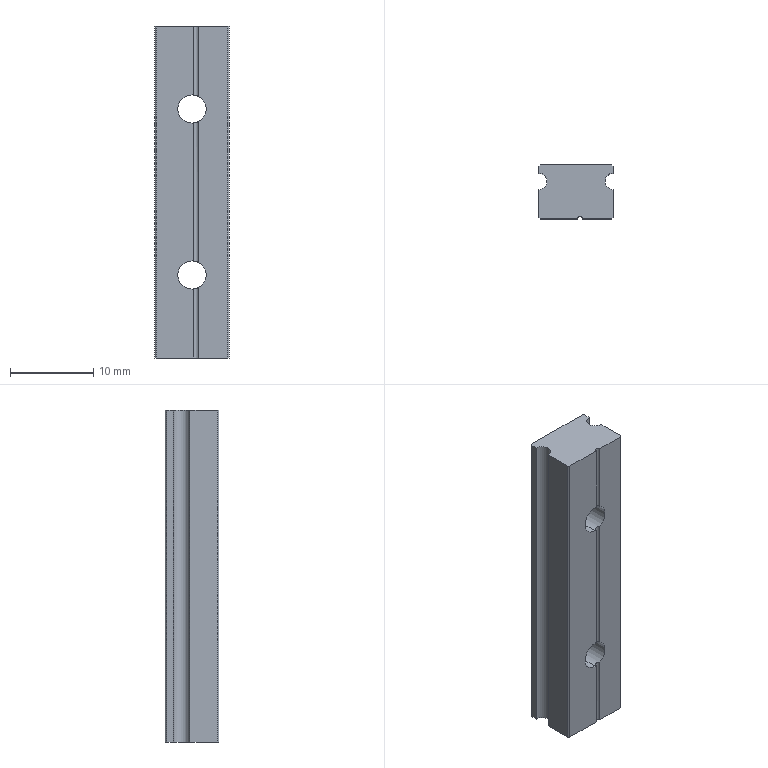Component | SolidWorks | MGN9C1R55Z0C(E=7.5)-10 | 1 solid | 29 faces | box 9 x 6.5 x 40 mm | volume 1924 mm3 | plane 15 | cylinder 14 | commonest cylinder face diameters 6.5 x4 3.4 x4 2 x3 0.6 x3
STEP:
#1=COLOUR_RGB('',0.7922,0.8196,0.9333);
#2=FILL_AREA_STYLE_COLOUR('',#1);
#3=FILL_AREA_STYLE('',(#2));
#4=SURFACE_STYLE_FILL_AREA(#3);
#5=SURFACE_SIDE_STYLE('',(#4));
#6=SURFACE_STYLE_USAGE(.BOTH.,#5);
#7=PRESENTATION_STYLE_ASSIGNMENT((#6));
#8=CARTESIAN_POINT('',(-1.043,-0.6806,-4.824));
#9=VERTEX_POINT('',#8);
#10=CARTESIAN_POINT('',(-1.043,-0.6806,-4.569));
#11=VERTEX_POINT('',#10);
#12=CARTESIAN_POINT('',(-1.043,-0.6806,-4.697));
#13=DIRECTION('',(0.,1.,0.));
#14=DIRECTION('',(0.,0.,1.));
#15=AXIS2_PLACEMENT_3D('',#12,#13,#14);
#16=CIRCLE('',#15,0.128);
#17=EDGE_CURVE('',#9,#11,#16,.T.);
#18=ORIENTED_EDGE('',*,*,#17,.F.);
#19=CARTESIAN_POINT('',(-1.043,-0.5468,-4.824));
#20=VERTEX_POINT('',#19);
#21=CARTESIAN_POINT('',(-1.043,-0.5468,-4.824));
#22=DIRECTION('',(0.,1.,0.));
#23=VECTOR('',#22,39.37);
#24=LINE('',#21,#23);
#25=EDGE_CURVE('',#9,#20,#24,.T.);
#26=ORIENTED_EDGE('',*,*,#25,.T.);
#27=CARTESIAN_POINT('',(-1.043,-0.5468,-4.569));
#28=VERTEX_POINT('',#27);
#29=CARTESIAN_POINT('',(-1.043,-0.5468,-4.697));
#30=DIRECTION('',(0.,1.,0.));
#31=DIRECTION('',(0.,0.,1.));
#32=AXIS2_PLACEMENT_3D('',#29,#30,#31);
#33=CIRCLE('',#32,0.128);
#34=EDGE_CURVE('',#20,#28,#33,.T.);
#35=ORIENTED_EDGE('',*,*,#34,.T.);
#36=CARTESIAN_POINT('',(-1.043,-0.5468,-4.569));
#37=DIRECTION('',(0.,1.,0.));
#38=VECTOR('',#37,39.37);
#39=LINE('',#36,#38);
#40=EDGE_CURVE('',#11,#28,#39,.T.);
#41=ORIENTED_EDGE('',*,*,#40,.F.);
#42=EDGE_LOOP('',(#18,#26,#35,#41));
#43=FACE_OUTER_BOUND('',#42,.T.);
#44=CARTESIAN_POINT('',(-1.043,-0.5468,-4.697));
#45=DIRECTION('',(0.,1.,0.));
#46=DIRECTION('',(0.,0.,1.));
#47=AXIS2_PLACEMENT_3D('',#44,#45,#46);
#48=CYLINDRICAL_SURFACE('',#47,0.128);
#49=ADVANCED_FACE('',(#43),#48,.F.);
#50=CARTESIAN_POINT('',(-1.043,-0.8027,-4.763));
#51=VERTEX_POINT('',#50);
#52=CARTESIAN_POINT('',(-1.043,-0.8027,-4.63));
#53=VERTEX_POINT('',#52);
#54=CARTESIAN_POINT('',(-1.043,-0.8027,-4.697));
#55=DIRECTION('',(-0.,1.,0.));
#56=DIRECTION('',(-1.,0.,0.));
#57=AXIS2_PLACEMENT_3D('',#54,#55,#56);
#58=CIRCLE('',#57,0.06693);
#59=EDGE_CURVE('',#51,#53,#58,.T.);
#60=ORIENTED_EDGE('',*,*,#59,.F.);
#61=CARTESIAN_POINT('',(-1.043,-0.6806,-4.763));
#62=VERTEX_POINT('',#61);
#63=CARTESIAN_POINT('',(-1.043,-0.5468,-4.763));
#64=DIRECTION('',(0.,1.,0.));
#65=VECTOR('',#64,39.37);
#66=LINE('',#63,#65);
#67=EDGE_CURVE('',#51,#62,#66,.T.);
#68=ORIENTED_EDGE('',*,*,#67,.T.);
#69=CARTESIAN_POINT('',(-1.043,-0.6806,-4.63));
#70=VERTEX_POINT('',#69);
#71=CARTESIAN_POINT('',(-1.043,-0.6806,-4.697));
#72=DIRECTION('',(0.,1.,0.));
#73=DIRECTION('',(0.,0.,1.));
#74=AXIS2_PLACEMENT_3D('',#71,#72,#73);
#75=CIRCLE('',#74,0.06693);
#76=EDGE_CURVE('',#62,#70,#75,.T.);
#77=ORIENTED_EDGE('',*,*,#76,.T.);
#78=CARTESIAN_POINT('',(-1.043,-0.5468,-4.63));
#79=DIRECTION('',(0.,1.,0.));
#80=VECTOR('',#79,39.37);
#81=LINE('',#78,#80);
#82=EDGE_CURVE('',#53,#70,#81,.T.);
#83=ORIENTED_EDGE('',*,*,#82,.F.);
#84=EDGE_LOOP('',(#60,#68,#77,#83));
#85=FACE_OUTER_BOUND('',#84,.T.);
#86=CARTESIAN_POINT('',(-1.043,-0.5468,-4.697));
#87=DIRECTION('',(0.,1.,0.));
#88=DIRECTION('',(0.,0.,1.));
#89=AXIS2_PLACEMENT_3D('',#86,#87,#88);
#90=CYLINDRICAL_SURFACE('',#89,0.06693);
#91=ADVANCED_FACE('',(#85),#90,.F.);
#92=CARTESIAN_POINT('',(-1.043,-0.6806,-4.037));
#93=VERTEX_POINT('',#92);
#94=CARTESIAN_POINT('',(-1.043,-0.6806,-3.781));
#95=VERTEX_POINT('',#94);
#96=CARTESIAN_POINT('',(-1.043,-0.6806,-3.909));
#97=DIRECTION('',(0.,1.,0.));
#98=DIRECTION('',(0.,0.,1.));
#99=AXIS2_PLACEMENT_3D('',#96,#97,#98);
#100=CIRCLE('',#99,0.128);
#101=EDGE_CURVE('',#93,#95,#100,.T.);
#102=ORIENTED_EDGE('',*,*,#101,.F.);
#103=CARTESIAN_POINT('',(-1.043,-0.5468,-4.037));
#104=VERTEX_POINT('',#103);
#105=CARTESIAN_POINT('',(-1.043,-0.5468,-4.037));
#106=DIRECTION('',(0.,1.,0.));
#107=VECTOR('',#106,39.37);
#108=LINE('',#105,#107);
#109=EDGE_CURVE('',#93,#104,#108,.T.);
#110=ORIENTED_EDGE('',*,*,#109,.T.);
#111=CARTESIAN_POINT('',(-1.043,-0.5468,-3.781));
#112=VERTEX_POINT('',#111);
#113=CARTESIAN_POINT('',(-1.043,-0.5468,-3.909));
#114=DIRECTION('',(0.,1.,0.));
#115=DIRECTION('',(0.,0.,1.));
#116=AXIS2_PLACEMENT_3D('',#113,#114,#115);
#117=CIRCLE('',#116,0.128);
#118=EDGE_CURVE('',#104,#112,#117,.T.);
#119=ORIENTED_EDGE('',*,*,#118,.T.);
#120=CARTESIAN_POINT('',(-1.043,-0.5468,-3.781));
#121=DIRECTION('',(0.,1.,0.));
#122=VECTOR('',#121,39.37);
#123=LINE('',#120,#122);
#124=EDGE_CURVE('',#95,#112,#123,.T.);
#125=ORIENTED_EDGE('',*,*,#124,.F.);
#126=EDGE_LOOP('',(#102,#110,#119,#125));
#127=FACE_OUTER_BOUND('',#126,.T.);
#128=CARTESIAN_POINT('',(-1.043,-0.5468,-3.909));
#129=DIRECTION('',(0.,1.,0.));
#130=DIRECTION('',(0.,0.,1.));
#131=AXIS2_PLACEMENT_3D('',#128,#129,#130);
#132=CYLINDRICAL_SURFACE('',#131,0.128);
#133=ADVANCED_FACE('',(#127),#132,.F.);
#134=CARTESIAN_POINT('',(-1.043,-0.8027,-3.976));
#135=VERTEX_POINT('',#134);
#136=CARTESIAN_POINT('',(-1.043,-0.8027,-3.842));
#137=VERTEX_POINT('',#136);
#138=CARTESIAN_POINT('',(-1.043,-0.8027,-3.909));
#139=DIRECTION('',(-0.,1.,0.));
#140=DIRECTION('',(-1.,0.,0.));
#141=AXIS2_PLACEMENT_3D('',#138,#139,#140);
#142=CIRCLE('',#141,0.06693);
#143=EDGE_CURVE('',#135,#137,#142,.T.);
#144=ORIENTED_EDGE('',*,*,#143,.F.);
#145=CARTESIAN_POINT('',(-1.043,-0.6806,-3.976));
#146=VERTEX_POINT('',#145);
#147=CARTESIAN_POINT('',(-1.043,-0.5468,-3.976));
#148=DIRECTION('',(0.,1.,0.));
#149=VECTOR('',#148,39.37);
#150=LINE('',#147,#149);
#151=EDGE_CURVE('',#135,#146,#150,.T.);
#152=ORIENTED_EDGE('',*,*,#151,.T.);
#153=CARTESIAN_POINT('',(-1.043,-0.6806,-3.842));
#154=VERTEX_POINT('',#153);
#155=CARTESIAN_POINT('',(-1.043,-0.6806,-3.909));
#156=DIRECTION('',(0.,1.,0.));
#157=DIRECTION('',(0.,0.,1.));
#158=AXIS2_PLACEMENT_3D('',#155,#156,#157);
#159=CIRCLE('',#158,0.06693);
#160=EDGE_CURVE('',#146,#154,#159,.T.);
#161=ORIENTED_EDGE('',*,*,#160,.T.);
#162=CARTESIAN_POINT('',(-1.043,-0.5468,-3.842));
#163=DIRECTION('',(0.,1.,0.));
#164=VECTOR('',#163,39.37);
#165=LINE('',#162,#164);
#166=EDGE_CURVE('',#137,#154,#165,.T.);
#167=ORIENTED_EDGE('',*,*,#166,.F.);
#168=EDGE_LOOP('',(#144,#152,#161,#167));
#169=FACE_OUTER_BOUND('',#168,.T.);
#170=CARTESIAN_POINT('',(-1.043,-0.5468,-3.909));
#171=DIRECTION('',(0.,1.,0.));
#172=DIRECTION('',(0.,0.,1.));
#173=AXIS2_PLACEMENT_3D('',#170,#171,#172);
#174=CYLINDRICAL_SURFACE('',#173,0.06693);
#175=ADVANCED_FACE('',(#169),#174,.F.);
#176=CARTESIAN_POINT('',(-0.8657,-0.5861,-3.515));
#177=VERTEX_POINT('',#176);
#178=CARTESIAN_POINT('',(-0.9051,-0.6255,-3.515));
#179=VERTEX_POINT('',#178);
#180=CARTESIAN_POINT('',(-0.8657,-0.6255,-3.515));
#181=DIRECTION('',(0.,0.,1.));
#182=DIRECTION('',(-1.,0.,0.));
#183=AXIS2_PLACEMENT_3D('',#180,#181,#182);
#184=CIRCLE('',#183,0.03937);
#185=EDGE_CURVE('',#177,#179,#184,.T.);
#186=ORIENTED_EDGE('',*,*,#185,.T.);
#187=CARTESIAN_POINT('',(-0.9051,-0.6255,-5.09));
#188=VERTEX_POINT('',#187);
#189=CARTESIAN_POINT('',(-0.9051,-0.6255,-3.515));
#190=DIRECTION('',(0.,0.,-1.));
#191=VECTOR('',#190,39.37);
#192=LINE('',#189,#191);
#193=EDGE_CURVE('',#179,#188,#192,.T.);
#194=ORIENTED_EDGE('',*,*,#193,.T.);
#195=CARTESIAN_POINT('',(-0.8657,-0.5861,-5.09));
#196=VERTEX_POINT('',#195);
#197=CARTESIAN_POINT('',(-0.8657,-0.6255,-5.09));
#198=DIRECTION('',(0.,0.,-1.));
#199=DIRECTION('',(1.,0.,0.));
#200=AXIS2_PLACEMENT_3D('',#197,#198,#199);
#201=CIRCLE('',#200,0.03937);
#202=EDGE_CURVE('',#188,#196,#201,.T.);
#203=ORIENTED_EDGE('',*,*,#202,.T.);
#204=CARTESIAN_POINT('',(-0.8657,-0.5861,-3.515));
#205=DIRECTION('',(0.,0.,-1.));
#206=VECTOR('',#205,39.37);
#207=LINE('',#204,#206);
#208=EDGE_CURVE('',#177,#196,#207,.T.);
#209=ORIENTED_EDGE('',*,*,#208,.F.);
#210=EDGE_LOOP('',(#186,#194,#203,#209));
#211=FACE_OUTER_BOUND('',#210,.T.);
#212=CARTESIAN_POINT('',(-0.8657,-0.6255,-3.515));
#213=DIRECTION('',(0.,0.,-1.));
#214=DIRECTION('',(-1.,0.,0.));
#215=AXIS2_PLACEMENT_3D('',#212,#213,#214);
#216=CYLINDRICAL_SURFACE('',#215,0.03937);
#217=ADVANCED_FACE('',(#211),#216,.F.);
#218=CARTESIAN_POINT('',(-1.035,-0.8027,-3.976));
#219=VERTEX_POINT('',#218);
#220=CARTESIAN_POINT('',(-1.035,-0.8027,-4.63));
#221=VERTEX_POINT('',#220);
#222=CARTESIAN_POINT('',(-1.035,-0.8027,-3.515));
#223=DIRECTION('',(0.,0.,-1.));
#224=VECTOR('',#223,39.37);
#225=LINE('',#222,#224);
#226=EDGE_CURVE('',#219,#221,#225,.T.);
#227=ORIENTED_EDGE('',*,*,#226,.T.);
#228=CARTESIAN_POINT('',(-1.011,-0.8027,-4.637));
#229=VERTEX_POINT('',#228);
#230=CARTESIAN_POINT('',(-1.035,-0.8027,-4.63));
#231=CARTESIAN_POINT('',(-1.035,-0.7995,-4.63));
#232=CARTESIAN_POINT('',(-1.034,-0.7963,-4.63));
#233=CARTESIAN_POINT('',(-1.029,-0.792,-4.631));
#234=CARTESIAN_POINT('',(-1.026,-0.7908,-4.632));
#235=CARTESIAN_POINT('',(-1.02,-0.7909,-4.634));
#236=CARTESIAN_POINT('',(-1.017,-0.7921,-4.635));
#237=CARTESIAN_POINT('',(-1.013,-0.7964,-4.637));
#238=CARTESIAN_POINT('',(-1.011,-0.7995,-4.637));
#239=CARTESIAN_POINT('',(-1.011,-0.8027,-4.637));
#240=B_SPLINE_CURVE_WITH_KNOTS('',3,(#230,#231,#232,#233,#234,#235,#236,#237,#238,#239),.UNSPECIFIED.,.F.,.F.,(4,2,2,2,4),(0.,0.0002407,0.0004815,0.0007222,0.0009629),.UNSPECIFIED.);
#241=EDGE_CURVE('',#221,#229,#240,.T.);
#242=ORIENTED_EDGE('',*,*,#241,.T.);
#243=CARTESIAN_POINT('',(-1.011,-0.8027,-3.968));
#244=VERTEX_POINT('',#243);
#245=CARTESIAN_POINT('',(-1.011,-0.8027,-3.515));
#246=DIRECTION('',(0.,0.,1.));
#247=VECTOR('',#246,39.37);
#248=LINE('',#245,#247);
#249=EDGE_CURVE('',#229,#244,#248,.T.);
#250=ORIENTED_EDGE('',*,*,#249,.T.);
#251=CARTESIAN_POINT('',(-1.011,-0.8027,-3.968));
#252=CARTESIAN_POINT('',(-1.011,-0.7995,-3.968));
#253=CARTESIAN_POINT('',(-1.013,-0.7964,-3.969));
#254=CARTESIAN_POINT('',(-1.017,-0.7922,-3.971));
#255=CARTESIAN_POINT('',(-1.02,-0.7909,-3.972));
#256=CARTESIAN_POINT('',(-1.026,-0.7908,-3.974));
#257=CARTESIAN_POINT('',(-1.029,-0.7919,-3.975));
#258=CARTESIAN_POINT('',(-1.034,-0.7963,-3.975));
#259=CARTESIAN_POINT('',(-1.035,-0.7995,-3.976));
#260=CARTESIAN_POINT('',(-1.035,-0.8027,-3.976));
#261=B_SPLINE_CURVE_WITH_KNOTS('',3,(#251,#252,#253,#254,#255,#256,#257,#258,#259,#260),.UNSPECIFIED.,.F.,.F.,(4,2,2,2,4),(0.,0.0002406,0.0004813,0.0007219,0.0009625),.UNSPECIFIED.);
#262=EDGE_CURVE('',#244,#219,#261,.T.);
#263=ORIENTED_EDGE('',*,*,#262,.T.);
#264=EDGE_LOOP('',(#227,#242,#250,#263));
#265=FACE_OUTER_BOUND('',#264,.T.);
#266=CARTESIAN_POINT('',(-1.023,-0.8027,-3.515));
#267=DIRECTION('',(0.,0.,-1.));
#268=DIRECTION('',(-1.,0.,0.));
#269=AXIS2_PLACEMENT_3D('',#266,#267,#268);
#270=CYLINDRICAL_SURFACE('',#269,0.01181);
#271=ADVANCED_FACE('',(#265),#270,.F.);
#272=CARTESIAN_POINT('',(-1.011,-0.8027,-5.09));
#273=VERTEX_POINT('',#272);
#274=CARTESIAN_POINT('',(-1.011,-0.8027,-4.756));
#275=VERTEX_POINT('',#274);
#276=CARTESIAN_POINT('',(-1.011,-0.8027,-3.515));
#277=DIRECTION('',(0.,0.,1.));
#278=VECTOR('',#277,39.37);
#279=LINE('',#276,#278);
#280=EDGE_CURVE('',#273,#275,#279,.T.);
#281=ORIENTED_EDGE('',*,*,#280,.T.);
#282=CARTESIAN_POINT('',(-1.035,-0.8027,-4.763));
#283=VERTEX_POINT('',#282);
#284=CARTESIAN_POINT('',(-1.011,-0.8027,-4.756));
#285=CARTESIAN_POINT('',(-1.011,-0.7995,-4.756));
#286=CARTESIAN_POINT('',(-1.013,-0.7964,-4.756));
#287=CARTESIAN_POINT('',(-1.017,-0.7922,-4.758));
#288=CARTESIAN_POINT('',(-1.02,-0.7909,-4.759));
#289=CARTESIAN_POINT('',(-1.026,-0.7908,-4.761));
#290=CARTESIAN_POINT('',(-1.029,-0.7919,-4.762));
#291=CARTESIAN_POINT('',(-1.034,-0.7963,-4.763));
#292=CARTESIAN_POINT('',(-1.035,-0.7995,-4.763));
#293=CARTESIAN_POINT('',(-1.035,-0.8027,-4.763));
#294=B_SPLINE_CURVE_WITH_KNOTS('',3,(#284,#285,#286,#287,#288,#289,#290,#291,#292,#293),.UNSPECIFIED.,.F.,.F.,(4,2,2,2,4),(0.,0.0002406,0.0004813,0.0007219,0.0009625),.UNSPECIFIED.);
#295=EDGE_CURVE('',#275,#283,#294,.T.);
#296=ORIENTED_EDGE('',*,*,#295,.T.);
#297=CARTESIAN_POINT('',(-1.035,-0.8027,-5.09));
#298=VERTEX_POINT('',#297);
#299=CARTESIAN_POINT('',(-1.035,-0.8027,-3.515));
#300=DIRECTION('',(0.,0.,-1.));
#301=VECTOR('',#300,39.37);
#302=LINE('',#299,#301);
#303=EDGE_CURVE('',#283,#298,#302,.T.);
#304=ORIENTED_EDGE('',*,*,#303,.T.);
#305=CARTESIAN_POINT('',(-1.023,-0.8027,-5.09));
#306=DIRECTION('',(0.,0.,-1.));
#307=DIRECTION('',(1.,0.,0.));
#308=AXIS2_PLACEMENT_3D('',#305,#306,#307);
#309=CIRCLE('',#308,0.01181);
#310=EDGE_CURVE('',#298,#273,#309,.T.);
#311=ORIENTED_EDGE('',*,*,#310,.T.);
#312=EDGE_LOOP('',(#281,#296,#304,#311));
#313=FACE_OUTER_BOUND('',#312,.T.);
#314=CARTESIAN_POINT('',(-1.023,-0.8027,-3.515));
#315=DIRECTION('',(0.,0.,-1.));
#316=DIRECTION('',(-1.,0.,0.));
#317=AXIS2_PLACEMENT_3D('',#314,#315,#316);
#318=CYLINDRICAL_SURFACE('',#317,0.01181);
#319=ADVANCED_FACE('',(#313),#318,.F.);
#320=CARTESIAN_POINT('',(-0.8736,-0.8027,-3.515));
#321=VERTEX_POINT('',#320);
#322=CARTESIAN_POINT('',(-0.8736,-0.8027,-5.09));
#323=VERTEX_POINT('',#322);
#324=CARTESIAN_POINT('',(-0.8736,-0.8027,-3.515));
#325=DIRECTION('',(0.,0.,-1.));
#326=VECTOR('',#325,39.37);
#327=LINE('',#324,#326);
#328=EDGE_CURVE('',#321,#323,#327,.T.);
#329=ORIENTED_EDGE('',*,*,#328,.T.);
#330=CARTESIAN_POINT('',(-0.8657,-0.7948,-5.09));
#331=VERTEX_POINT('',#330);
#332=CARTESIAN_POINT('',(-0.8736,-0.8027,-5.09));
#333=DIRECTION('',(0.7071,0.7071,0.));
#334=VECTOR('',#333,39.37);
#335=LINE('',#332,#334);
#336=EDGE_CURVE('',#323,#331,#335,.T.);
#337=ORIENTED_EDGE('',*,*,#336,.T.);
#338=CARTESIAN_POINT('',(-0.8657,-0.7948,-3.515));
#339=VERTEX_POINT('',#338);
#340=CARTESIAN_POINT('',(-0.8657,-0.7948,-3.515));
#341=DIRECTION('',(0.,0.,1.));
#342=VECTOR('',#341,39.37);
#343=LINE('',#340,#342);
#344=EDGE_CURVE('',#331,#339,#343,.T.);
#345=ORIENTED_EDGE('',*,*,#344,.T.);
#346=CARTESIAN_POINT('',(-0.8657,-0.7948,-3.515));
#347=DIRECTION('',(0.7071,0.7071,0.));
#348=VECTOR('',#347,39.37);
#349=LINE('',#346,#348);
#350=EDGE_CURVE('',#321,#339,#349,.T.);
#351=ORIENTED_EDGE('',*,*,#350,.F.);
#352=EDGE_LOOP('',(#329,#337,#345,#351));
#353=FACE_OUTER_BOUND('',#352,.T.);
#354=CARTESIAN_POINT('',(-0.8657,-0.7948,-3.515));
#355=DIRECTION('',(-0.7071,0.7071,0.));
#356=DIRECTION('',(-0.7071,-0.7071,0.));
#357=AXIS2_PLACEMENT_3D('',#354,#355,#356);
#358=PLANE('',#357);
#359=ADVANCED_FACE('',(#353),#358,.F.);
#360=CARTESIAN_POINT('',(-1.035,-0.8027,-3.515));
#361=VERTEX_POINT('',#360);
#362=CARTESIAN_POINT('',(-1.035,-0.8027,-3.843));
#363=VERTEX_POINT('',#362);
#364=CARTESIAN_POINT('',(-1.035,-0.8027,-3.515));
#365=DIRECTION('',(0.,0.,-1.));
#366=VECTOR('',#365,39.37);
#367=LINE('',#364,#366);
#368=EDGE_CURVE('',#361,#363,#367,.T.);
#369=ORIENTED_EDGE('',*,*,#368,.T.);
#370=CARTESIAN_POINT('',(-1.011,-0.8027,-3.85));
#371=VERTEX_POINT('',#370);
#372=CARTESIAN_POINT('',(-1.035,-0.8027,-3.843));
#373=CARTESIAN_POINT('',(-1.035,-0.7995,-3.843));
#374=CARTESIAN_POINT('',(-1.034,-0.7963,-3.843));
#375=CARTESIAN_POINT('',(-1.029,-0.792,-3.844));
#376=CARTESIAN_POINT('',(-1.026,-0.7908,-3.844));
#377=CARTESIAN_POINT('',(-1.02,-0.7909,-3.846));
#378=CARTESIAN_POINT('',(-1.017,-0.7921,-3.847));
#379=CARTESIAN_POINT('',(-1.013,-0.7964,-3.849));
#380=CARTESIAN_POINT('',(-1.011,-0.7995,-3.85));
#381=CARTESIAN_POINT('',(-1.011,-0.8027,-3.85));
#382=B_SPLINE_CURVE_WITH_KNOTS('',3,(#372,#373,#374,#375,#376,#377,#378,#379,#380,#381),.UNSPECIFIED.,.F.,.F.,(4,2,2,2,4),(0.,0.0002407,0.0004815,0.0007222,0.0009629),.UNSPECIFIED.);
#383=EDGE_CURVE('',#363,#371,#382,.T.);
#384=ORIENTED_EDGE('',*,*,#383,.T.);
#385=CARTESIAN_POINT('',(-1.011,-0.8027,-3.515));
#386=VERTEX_POINT('',#385);
#387=CARTESIAN_POINT('',(-1.011,-0.8027,-3.515));
#388=DIRECTION('',(0.,0.,1.));
#389=VECTOR('',#388,39.37);
#390=LINE('',#387,#389);
#391=EDGE_CURVE('',#371,#386,#390,.T.);
#392=ORIENTED_EDGE('',*,*,#391,.T.);
#393=CARTESIAN_POINT('',(-1.023,-0.8027,-3.515));
#394=DIRECTION('',(0.,0.,-1.));
#395=DIRECTION('',(-1.,0.,0.));
#396=AXIS2_PLACEMENT_3D('',#393,#394,#395);
#397=CIRCLE('',#396,0.01181);
#398=EDGE_CURVE('',#361,#386,#397,.T.);
#399=ORIENTED_EDGE('',*,*,#398,.F.);
#400=EDGE_LOOP('',(#369,#384,#392,#399));
#401=FACE_OUTER_BOUND('',#400,.T.);
#402=CARTESIAN_POINT('',(-1.023,-0.8027,-3.515));
#403=DIRECTION('',(0.,0.,-1.));
#404=DIRECTION('',(-1.,0.,0.));
#405=AXIS2_PLACEMENT_3D('',#402,#403,#404);
#406=CYLINDRICAL_SURFACE('',#405,0.01181);
#407=ADVANCED_FACE('',(#401),#406,.F.);
#408=CARTESIAN_POINT('',(-1.22,-0.7948,-3.515));
#409=VERTEX_POINT('',#408);
#410=CARTESIAN_POINT('',(-1.22,-0.7948,-5.09));
#411=VERTEX_POINT('',#410);
#412=CARTESIAN_POINT('',(-1.22,-0.7948,-3.515));
#413=DIRECTION('',(0.,0.,-1.));
#414=VECTOR('',#413,39.37);
#415=LINE('',#412,#414);
#416=EDGE_CURVE('',#409,#411,#415,.T.);
#417=ORIENTED_EDGE('',*,*,#416,.T.);
#418=CARTESIAN_POINT('',(-1.212,-0.8027,-5.09));
#419=VERTEX_POINT('',#418);
#420=CARTESIAN_POINT('',(-1.22,-0.7948,-5.09));
#421=DIRECTION('',(0.7071,-0.7071,0.));
#422=VECTOR('',#421,39.37);
#423=LINE('',#420,#422);
#424=EDGE_CURVE('',#411,#419,#423,.T.);
#425=ORIENTED_EDGE('',*,*,#424,.T.);
#426=CARTESIAN_POINT('',(-1.212,-0.8027,-3.515));
#427=VERTEX_POINT('',#426);
#428=CARTESIAN_POINT('',(-1.212,-0.8027,-3.515));
#429=DIRECTION('',(0.,0.,1.));
#430=VECTOR('',#429,39.37);
#431=LINE('',#428,#430);
#432=EDGE_CURVE('',#419,#427,#431,.T.);
#433=ORIENTED_EDGE('',*,*,#432,.T.);
#434=CARTESIAN_POINT('',(-1.212,-0.8027,-3.515));
#435=DIRECTION('',(0.7071,-0.7071,0.));
#436=VECTOR('',#435,39.37);
#437=LINE('',#434,#436);
#438=EDGE_CURVE('',#409,#427,#437,.T.);
#439=ORIENTED_EDGE('',*,*,#438,.F.);
#440=EDGE_LOOP('',(#417,#425,#433,#439));
#441=FACE_OUTER_BOUND('',#440,.T.);
#442=CARTESIAN_POINT('',(-1.212,-0.8027,-3.515));
#443=DIRECTION('',(0.7071,0.7071,0.));
#444=DIRECTION('',(-0.7071,0.7071,0.));
#445=AXIS2_PLACEMENT_3D('',#442,#443,#444);
#446=PLANE('',#445);
#447=ADVANCED_FACE('',(#441),#446,.F.);
#448=ORIENTED_EDGE('',*,*,#208,.T.);
#449=CARTESIAN_POINT('',(-0.8657,-0.5546,-5.09));
#450=VERTEX_POINT('',#449);
#451=CARTESIAN_POINT('',(-0.8657,-0.5861,-5.09));
#452=DIRECTION('',(0.,1.,0.));
#453=VECTOR('',#452,39.37);
#454=LINE('',#451,#453);
#455=EDGE_CURVE('',#196,#450,#454,.T.);
#456=ORIENTED_EDGE('',*,*,#455,.T.);
#457=CARTESIAN_POINT('',(-0.8657,-0.5546,-3.515));
#458=VERTEX_POINT('',#457);
#459=CARTESIAN_POINT('',(-0.8657,-0.5546,-3.515));
#460=DIRECTION('',(0.,0.,1.));
#461=VECTOR('',#460,39.37);
#462=LINE('',#459,#461);
#463=EDGE_CURVE('',#450,#458,#462,.T.);
#464=ORIENTED_EDGE('',*,*,#463,.T.);
#465=CARTESIAN_POINT('',(-0.8657,-0.5861,-3.515));
#466=DIRECTION('',(0.,1.,0.));
#467=VECTOR('',#466,39.37);
#468=LINE('',#465,#467);
#469=EDGE_CURVE('',#177,#458,#468,.T.);
#470=ORIENTED_EDGE('',*,*,#469,.F.);
#471=EDGE_LOOP('',(#448,#456,#464,#470));
#472=FACE_OUTER_BOUND('',#471,.T.);
#473=CARTESIAN_POINT('',(-0.8657,-0.5861,-3.515));
#474=DIRECTION('',(-1.,0.,0.));
#475=DIRECTION('',(0.,0.,1.));
#476=AXIS2_PLACEMENT_3D('',#473,#474,#475);
#477=PLANE('',#476);
#478=ADVANCED_FACE('',(#472),#477,.F.);
#479=CARTESIAN_POINT('',(-1.22,-0.5546,-3.515));
#480=VERTEX_POINT('',#479);
#481=CARTESIAN_POINT('',(-1.22,-0.5546,-5.09));
#482=VERTEX_POINT('',#481);
#483=CARTESIAN_POINT('',(-1.22,-0.5546,-3.515));
#484=DIRECTION('',(0.,0.,-1.));
#485=VECTOR('',#484,39.37);
#486=LINE('',#483,#485);
#487=EDGE_CURVE('',#480,#482,#486,.T.);
#488=ORIENTED_EDGE('',*,*,#487,.T.);
#489=CARTESIAN_POINT('',(-1.22,-0.5861,-5.09));
#490=VERTEX_POINT('',#489);
#491=CARTESIAN_POINT('',(-1.22,-0.5546,-5.09));
#492=DIRECTION('',(0.,-1.,0.));
#493=VECTOR('',#492,39.37);
#494=LINE('',#491,#493);
#495=EDGE_CURVE('',#482,#490,#494,.T.);
#496=ORIENTED_EDGE('',*,*,#495,.T.);
#497=CARTESIAN_POINT('',(-1.22,-0.5861,-3.515));
#498=VERTEX_POINT('',#497);
#499=CARTESIAN_POINT('',(-1.22,-0.5861,-3.515));
#500=DIRECTION('',(0.,0.,1.));
#501=VECTOR('',#500,39.37);
#502=LINE('',#499,#501);
#503=EDGE_CURVE('',#490,#498,#502,.T.);
#504=ORIENTED_EDGE('',*,*,#503,.T.);
#505=CARTESIAN_POINT('',(-1.22,-0.8027,-3.515));
#506=DIRECTION('',(0.,1.,0.));
#507=VECTOR('',#506,39.37);
#508=LINE('',#505,#507);
#509=EDGE_CURVE('',#498,#480,#508,.T.);
#510=ORIENTED_EDGE('',*,*,#509,.T.);
#511=EDGE_LOOP('',(#488,#496,#504,#510));
#512=FACE_OUTER_BOUND('',#511,.T.);
#513=CARTESIAN_POINT('',(-1.22,-0.5468,-3.515));
#514=DIRECTION('',(1.,0.,0.));
#515=DIRECTION('',(0.,0.,-1.));
#516=AXIS2_PLACEMENT_3D('',#513,#514,#515);
#517=PLANE('',#516);
#518=ADVANCED_FACE('',(#512),#517,.F.);
#519=ORIENTED_EDGE('',*,*,#344,.F.);
#520=CARTESIAN_POINT('',(-0.8657,-0.6649,-5.09));
#521=VERTEX_POINT('',#520);
#522=CARTESIAN_POINT('',(-0.8657,-0.7948,-5.09));
#523=DIRECTION('',(0.,1.,0.));
#524=VECTOR('',#523,39.37);
#525=LINE('',#522,#524);
#526=EDGE_CURVE('',#331,#521,#525,.T.);
#527=ORIENTED_EDGE('',*,*,#526,.T.);
#528=CARTESIAN_POINT('',(-0.8657,-0.6649,-3.515));
#529=VERTEX_POINT('',#528);
#530=CARTESIAN_POINT('',(-0.8657,-0.6649,-3.515));
#531=DIRECTION('',(0.,0.,1.));
#532=VECTOR('',#531,39.37);
#533=LINE('',#530,#532);
#534=EDGE_CURVE('',#521,#529,#533,.T.);
#535=ORIENTED_EDGE('',*,*,#534,.T.);
#536=CARTESIAN_POINT('',(-0.8657,-0.8027,-3.515));
#537=DIRECTION('',(0.,-1.,0.));
#538=VECTOR('',#537,39.37);
#539=LINE('',#536,#538);
#540=EDGE_CURVE('',#529,#339,#539,.T.);
#541=ORIENTED_EDGE('',*,*,#540,.T.);
#542=EDGE_LOOP('',(#519,#527,#535,#541));
#543=FACE_OUTER_BOUND('',#542,.T.);
#544=CARTESIAN_POINT('',(-0.8657,-0.8027,-3.515));
#545=DIRECTION('',(-1.,-0.,0.));
#546=DIRECTION('',(0.,-1.,0.));
#547=AXIS2_PLACEMENT_3D('',#544,#545,#546);
#548=PLANE('',#547);
#549=ADVANCED_FACE('',(#543),#548,.F.);
#550=ORIENTED_EDGE('',*,*,#249,.F.);
#551=CARTESIAN_POINT('',(-1.043,-0.8027,-4.697));
#552=DIRECTION('',(-0.,1.,0.));
#553=DIRECTION('',(-1.,0.,0.));
#554=AXIS2_PLACEMENT_3D('',#551,#552,#553);
#555=CIRCLE('',#554,0.06693);
#556=EDGE_CURVE('',#229,#275,#555,.T.);
#557=ORIENTED_EDGE('',*,*,#556,.T.);
#558=ORIENTED_EDGE('',*,*,#280,.F.);
#559=CARTESIAN_POINT('',(-1.011,-0.8027,-5.09));
#560=DIRECTION('',(1.,0.,0.));
#561=VECTOR('',#560,39.37);
#562=LINE('',#559,#561);
#563=EDGE_CURVE('',#273,#323,#562,.T.);
#564=ORIENTED_EDGE('',*,*,#563,.T.);
#565=ORIENTED_EDGE('',*,*,#328,.F.);
#566=CARTESIAN_POINT('',(-1.023,-0.8027,-3.515));
#567=DIRECTION('',(-1.,0.,0.));
#568=VECTOR('',#567,39.37);
#569=LINE('',#566,#568);
#570=EDGE_CURVE('',#321,#386,#569,.T.);
#571=ORIENTED_EDGE('',*,*,#570,.T.);
#572=ORIENTED_EDGE('',*,*,#391,.F.);
#573=CARTESIAN_POINT('',(-1.043,-0.8027,-3.909));
#574=DIRECTION('',(-0.,1.,0.));
#575=DIRECTION('',(-1.,0.,0.));
#576=AXIS2_PLACEMENT_3D('',#573,#574,#575);
#577=CIRCLE('',#576,0.06693);
#578=EDGE_CURVE('',#371,#244,#577,.T.);
#579=ORIENTED_EDGE('',*,*,#578,.T.);
#580=EDGE_LOOP('',(#550,#557,#558,#564,#565,#571,#572,#579));
#581=FACE_OUTER_BOUND('',#580,.T.);
#582=CARTESIAN_POINT('',(-1.011,-0.8027,-3.515));
#583=DIRECTION('',(-0.,1.,0.));
#584=DIRECTION('',(-1.,-0.,0.));
#585=AXIS2_PLACEMENT_3D('',#582,#583,#584);
#586=PLANE('',#585);
#587=ADVANCED_FACE('',(#581),#586,.F.);
#588=ORIENTED_EDGE('',*,*,#303,.F.);
#589=CARTESIAN_POINT('',(-1.043,-0.8027,-4.697));
#590=DIRECTION('',(-0.,1.,0.));
#591=DIRECTION('',(-1.,0.,0.));
#592=AXIS2_PLACEMENT_3D('',#589,#590,#591);
#593=CIRCLE('',#592,0.06693);
#594=EDGE_CURVE('',#283,#51,#593,.T.);
#595=ORIENTED_EDGE('',*,*,#594,.T.);
#596=ORIENTED_EDGE('',*,*,#59,.T.);
#597=CARTESIAN_POINT('',(-1.043,-0.8027,-4.697));
#598=DIRECTION('',(-0.,1.,0.));
#599=DIRECTION('',(-1.,0.,0.));
#600=AXIS2_PLACEMENT_3D('',#597,#598,#599);
#601=CIRCLE('',#600,0.06693);
#602=EDGE_CURVE('',#53,#221,#601,.T.);
#603=ORIENTED_EDGE('',*,*,#602,.T.);
#604=ORIENTED_EDGE('',*,*,#226,.F.);
#605=CARTESIAN_POINT('',(-1.043,-0.8027,-3.909));
#606=DIRECTION('',(-0.,1.,0.));
#607=DIRECTION('',(-1.,0.,0.));
#608=AXIS2_PLACEMENT_3D('',#605,#606,#607);
#609=CIRCLE('',#608,0.06693);
#610=EDGE_CURVE('',#219,#135,#609,.T.);
#611=ORIENTED_EDGE('',*,*,#610,.T.);
#612=ORIENTED_EDGE('',*,*,#143,.T.);
#613=CARTESIAN_POINT('',(-1.043,-0.8027,-3.909));
#614=DIRECTION('',(-0.,1.,0.));
#615=DIRECTION('',(-1.,0.,0.));
#616=AXIS2_PLACEMENT_3D('',#613,#614,#615);
#617=CIRCLE('',#616,0.06693);
#618=EDGE_CURVE('',#137,#363,#617,.T.);
#619=ORIENTED_EDGE('',*,*,#618,.T.);
#620=ORIENTED_EDGE('',*,*,#368,.F.);
#621=CARTESIAN_POINT('',(-1.023,-0.8027,-3.515));
#622=DIRECTION('',(-1.,0.,0.));
#623=VECTOR('',#622,39.37);
#624=LINE('',#621,#623);
#625=EDGE_CURVE('',#361,#427,#624,.T.);
#626=ORIENTED_EDGE('',*,*,#625,.T.);
#627=ORIENTED_EDGE('',*,*,#432,.F.);
#628=CARTESIAN_POINT('',(-1.212,-0.8027,-5.09));
#629=DIRECTION('',(1.,0.,0.));
#630=VECTOR('',#629,39.37);
#631=LINE('',#628,#630);
#632=EDGE_CURVE('',#419,#298,#631,.T.);
#633=ORIENTED_EDGE('',*,*,#632,.T.);
#634=EDGE_LOOP('',(#588,#595,#596,#603,#604,#611,#612,#619,#620,#626,#627,#633));
#635=FACE_OUTER_BOUND('',#634,.T.);
#636=CARTESIAN_POINT('',(-1.22,-0.8027,-3.515));
#637=DIRECTION('',(-0.,1.,0.));
#638=DIRECTION('',(-1.,-0.,0.));
#639=AXIS2_PLACEMENT_3D('',#636,#637,#638);
#640=PLANE('',#639);
#641=ADVANCED_FACE('',(#635),#640,.F.);
#642=CARTESIAN_POINT('',(-1.22,-0.6649,-3.515));
#643=VERTEX_POINT('',#642);
#644=CARTESIAN_POINT('',(-1.22,-0.6649,-5.09));
#645=VERTEX_POINT('',#644);
#646=CARTESIAN_POINT('',(-1.22,-0.6649,-3.515));
#647=DIRECTION('',(0.,0.,-1.));
#648=VECTOR('',#647,39.37);
#649=LINE('',#646,#648);
#650=EDGE_CURVE('',#643,#645,#649,.T.);
#651=ORIENTED_EDGE('',*,*,#650,.T.);
#652=CARTESIAN_POINT('',(-1.22,-0.6649,-5.09));
#653=DIRECTION('',(0.,-1.,0.));
#654=VECTOR('',#653,39.37);
#655=LINE('',#652,#654);
#656=EDGE_CURVE('',#645,#411,#655,.T.);
#657=ORIENTED_EDGE('',*,*,#656,.T.);
#658=ORIENTED_EDGE('',*,*,#416,.F.);
#659=CARTESIAN_POINT('',(-1.22,-0.8027,-3.515));
#660=DIRECTION('',(0.,1.,0.));
#661=VECTOR('',#660,39.37);
#662=LINE('',#659,#661);
#663=EDGE_CURVE('',#409,#643,#662,.T.);
#664=ORIENTED_EDGE('',*,*,#663,.T.);
#665=EDGE_LOOP('',(#651,#657,#658,#664));
#666=FACE_OUTER_BOUND('',#665,.T.);
#667=CARTESIAN_POINT('',(-1.22,-0.6649,-3.515));
#668=DIRECTION('',(1.,0.,0.));
#669=DIRECTION('',(-0.,1.,0.));
#670=AXIS2_PLACEMENT_3D('',#667,#668,#669);
#671=PLANE('',#670);
#672=ADVANCED_FACE('',(#666),#671,.F.);
#673=ORIENTED_EDGE('',*,*,#503,.F.);
#674=CARTESIAN_POINT('',(-1.22,-0.6255,-5.09));
#675=DIRECTION('',(0.,0.,-1.));
#676=DIRECTION('',(1.,0.,0.));
#677=AXIS2_PLACEMENT_3D('',#674,#675,#676);
#678=CIRCLE('',#677,0.03937);
#679=EDGE_CURVE('',#490,#645,#678,.T.);
#680=ORIENTED_EDGE('',*,*,#679,.T.);
#681=ORIENTED_EDGE('',*,*,#650,.F.);
#682=CARTESIAN_POINT('',(-1.22,-0.6255,-3.515));
#683=DIRECTION('',(0.,0.,1.));
#684=DIRECTION('',(-1.,0.,0.));
#685=AXIS2_PLACEMENT_3D('',#682,#683,#684);
#686=CIRCLE('',#685,0.03937);
#687=EDGE_CURVE('',#643,#498,#686,.T.);
#688=ORIENTED_EDGE('',*,*,#687,.T.);
#689=EDGE_LOOP('',(#673,#680,#681,#688));
#690=FACE_OUTER_BOUND('',#689,.T.);
#691=CARTESIAN_POINT('',(-1.22,-0.6255,-3.515));
#692=DIRECTION('',(0.,0.,-1.));
#693=DIRECTION('',(-1.,0.,0.));
#694=AXIS2_PLACEMENT_3D('',#691,#692,#693);
#695=CYLINDRICAL_SURFACE('',#694,0.03937);
#696=ADVANCED_FACE('',(#690),#695,.F.);
#697=ORIENTED_EDGE('',*,*,#193,.F.);
#698=CARTESIAN_POINT('',(-0.8657,-0.6255,-3.515));
#699=DIRECTION('',(0.,0.,1.));
#700=DIRECTION('',(-1.,0.,0.));
#701=AXIS2_PLACEMENT_3D('',#698,#699,#700);
#702=CIRCLE('',#701,0.03937);
#703=EDGE_CURVE('',#179,#529,#702,.T.);
#704=ORIENTED_EDGE('',*,*,#703,.T.);
#705=ORIENTED_EDGE('',*,*,#534,.F.);
#706=CARTESIAN_POINT('',(-0.8657,-0.6255,-5.09));
#707=DIRECTION('',(0.,0.,-1.));
#708=DIRECTION('',(1.,0.,0.));
#709=AXIS2_PLACEMENT_3D('',#706,#707,#708);
#710=CIRCLE('',#709,0.03937);
#711=EDGE_CURVE('',#521,#188,#710,.T.);
#712=ORIENTED_EDGE('',*,*,#711,.T.);
#713=EDGE_LOOP('',(#697,#704,#705,#712));
#714=FACE_OUTER_BOUND('',#713,.T.);
#715=CARTESIAN_POINT('',(-0.8657,-0.6255,-3.515));
#716=DIRECTION('',(0.,0.,-1.));
#717=DIRECTION('',(-1.,0.,0.));
#718=AXIS2_PLACEMENT_3D('',#715,#716,#717);
#719=CYLINDRICAL_SURFACE('',#718,0.03937);
#720=ADVANCED_FACE('',(#714),#719,.F.);
#721=ORIENTED_EDGE('',*,*,#463,.F.);
#722=CARTESIAN_POINT('',(-0.8736,-0.5468,-5.09));
#723=VERTEX_POINT('',#722);
#724=CARTESIAN_POINT('',(-0.8657,-0.5546,-5.09));
#725=DIRECTION('',(-0.7071,0.7071,0.));
#726=VECTOR('',#725,39.37);
#727=LINE('',#724,#726);
#728=EDGE_CURVE('',#450,#723,#727,.T.);
#729=ORIENTED_EDGE('',*,*,#728,.T.);
#730=CARTESIAN_POINT('',(-0.8736,-0.5468,-3.515));
#731=VERTEX_POINT('',#730);
#732=CARTESIAN_POINT('',(-0.8736,-0.5468,-3.515));
#733=DIRECTION('',(0.,0.,1.));
#734=VECTOR('',#733,39.37);
#735=LINE('',#732,#734);
#736=EDGE_CURVE('',#723,#731,#735,.T.);
#737=ORIENTED_EDGE('',*,*,#736,.T.);
#738=CARTESIAN_POINT('',(-0.8736,-0.5468,-3.515));
#739=DIRECTION('',(0.7071,-0.7071,0.));
#740=VECTOR('',#739,39.37);
#741=LINE('',#738,#740);
#742=EDGE_CURVE('',#731,#458,#741,.T.);
#743=ORIENTED_EDGE('',*,*,#742,.T.);
#744=EDGE_LOOP('',(#721,#729,#737,#743));
#745=FACE_OUTER_BOUND('',#744,.T.);
#746=CARTESIAN_POINT('',(-0.8736,-0.5468,-3.515));
#747=DIRECTION('',(-0.7071,-0.7071,0.));
#748=DIRECTION('',(0.7071,-0.7071,0.));
#749=AXIS2_PLACEMENT_3D('',#746,#747,#748);
#750=PLANE('',#749);
#751=ADVANCED_FACE('',(#745),#750,.F.);
#752=CARTESIAN_POINT('',(-1.212,-0.5468,-3.515));
#753=VERTEX_POINT('',#752);
#754=CARTESIAN_POINT('',(-1.212,-0.5468,-5.09));
#755=VERTEX_POINT('',#754);
#756=CARTESIAN_POINT('',(-1.212,-0.5468,-3.515));
#757=DIRECTION('',(0.,0.,-1.));
#758=VECTOR('',#757,39.37);
#759=LINE('',#756,#758);
#760=EDGE_CURVE('',#753,#755,#759,.T.);
#761=ORIENTED_EDGE('',*,*,#760,.T.);
#762=CARTESIAN_POINT('',(-1.212,-0.5468,-5.09));
#763=DIRECTION('',(-0.7071,-0.7071,0.));
#764=VECTOR('',#763,39.37);
#765=LINE('',#762,#764);
#766=EDGE_CURVE('',#755,#482,#765,.T.);
#767=ORIENTED_EDGE('',*,*,#766,.T.);
#768=ORIENTED_EDGE('',*,*,#487,.F.);
#769=CARTESIAN_POINT('',(-1.22,-0.5546,-3.515));
#770=DIRECTION('',(-0.7071,-0.7071,0.));
#771=VECTOR('',#770,39.37);
#772=LINE('',#769,#771);
#773=EDGE_CURVE('',#753,#480,#772,.T.);
#774=ORIENTED_EDGE('',*,*,#773,.F.);
#775=EDGE_LOOP('',(#761,#767,#768,#774));
#776=FACE_OUTER_BOUND('',#775,.T.);
#777=CARTESIAN_POINT('',(-1.22,-0.5546,-3.515));
#778=DIRECTION('',(0.7071,-0.7071,0.));
#779=DIRECTION('',(0.7071,0.7071,0.));
#780=AXIS2_PLACEMENT_3D('',#777,#778,#779);
#781=PLANE('',#780);
#782=ADVANCED_FACE('',(#776),#781,.F.);
#783=CARTESIAN_POINT('',(-1.043,-0.5468,-4.697));
#784=DIRECTION('',(0.,1.,0.));
#785=DIRECTION('',(0.,0.,1.));
#786=AXIS2_PLACEMENT_3D('',#783,#784,#785);
#787=CIRCLE('',#786,0.128);
#788=EDGE_CURVE('',#28,#20,#787,.T.);
#789=ORIENTED_EDGE('',*,*,#788,.F.);
#790=ORIENTED_EDGE('',*,*,#34,.F.);
#791=EDGE_LOOP('',(#789,#790));
#792=FACE_BOUND('',#791,.T.);
#793=CARTESIAN_POINT('',(-1.043,-0.5468,-3.909));
#794=DIRECTION('',(0.,1.,0.));
#795=DIRECTION('',(0.,0.,1.));
#796=AXIS2_PLACEMENT_3D('',#793,#794,#795);
#797=CIRCLE('',#796,0.128);
#798=EDGE_CURVE('',#112,#104,#797,.T.);
#799=ORIENTED_EDGE('',*,*,#798,.F.);
#800=ORIENTED_EDGE('',*,*,#118,.F.);
#801=EDGE_LOOP('',(#799,#800));
#802=FACE_BOUND('',#801,.T.);
#803=ORIENTED_EDGE('',*,*,#736,.F.);
#804=CARTESIAN_POINT('',(-0.8736,-0.5468,-5.09));
#805=DIRECTION('',(-1.,0.,0.));
#806=VECTOR('',#805,39.37);
#807=LINE('',#804,#806);
#808=EDGE_CURVE('',#723,#755,#807,.T.);
#809=ORIENTED_EDGE('',*,*,#808,.T.);
#810=ORIENTED_EDGE('',*,*,#760,.F.);
#811=CARTESIAN_POINT('',(-0.8657,-0.5468,-3.515));
#812=DIRECTION('',(-1.,0.,0.));
#813=VECTOR('',#812,39.37);
#814=LINE('',#811,#813);
#815=EDGE_CURVE('',#731,#753,#814,.T.);
#816=ORIENTED_EDGE('',*,*,#815,.F.);
#817=EDGE_LOOP('',(#803,#809,#810,#816));
#818=FACE_OUTER_BOUND('',#817,.T.);
#819=CARTESIAN_POINT('',(-0.8657,-0.5468,-3.515));
#820=DIRECTION('',(0.,-1.,0.));
#821=DIRECTION('',(0.,0.,-1.));
#822=AXIS2_PLACEMENT_3D('',#819,#820,#821);
#823=PLANE('',#822);
#824=ADVANCED_FACE('',(#792,#802,#818),#823,.F.);
#825=ORIENTED_EDGE('',*,*,#350,.T.);
#826=ORIENTED_EDGE('',*,*,#540,.F.);
#827=ORIENTED_EDGE('',*,*,#703,.F.);
#828=ORIENTED_EDGE('',*,*,#185,.F.);
#829=ORIENTED_EDGE('',*,*,#469,.T.);
#830=ORIENTED_EDGE('',*,*,#742,.F.);
#831=ORIENTED_EDGE('',*,*,#815,.T.);
#832=ORIENTED_EDGE('',*,*,#773,.T.);
#833=ORIENTED_EDGE('',*,*,#509,.F.);
#834=ORIENTED_EDGE('',*,*,#687,.F.);
#835=ORIENTED_EDGE('',*,*,#663,.F.);
#836=ORIENTED_EDGE('',*,*,#438,.T.);
#837=ORIENTED_EDGE('',*,*,#625,.F.);
#838=ORIENTED_EDGE('',*,*,#398,.T.);
#839=ORIENTED_EDGE('',*,*,#570,.F.);
#840=EDGE_LOOP('',(#825,#826,#827,#828,#829,#830,#831,#832,#833,#834,#835,#836,#837,#838,#839));
#841=FACE_OUTER_BOUND('',#840,.T.);
#842=CARTESIAN_POINT('',(-1.023,-0.8027,-3.515));
#843=DIRECTION('',(0.,0.,-1.));
#844=DIRECTION('',(-1.,0.,0.));
#845=AXIS2_PLACEMENT_3D('',#842,#843,#844);
#846=PLANE('',#845);
#847=ADVANCED_FACE('',(#841),#846,.F.);
#848=ORIENTED_EDGE('',*,*,#563,.F.);
#849=ORIENTED_EDGE('',*,*,#310,.F.);
#850=ORIENTED_EDGE('',*,*,#632,.F.);
#851=ORIENTED_EDGE('',*,*,#424,.F.);
#852=ORIENTED_EDGE('',*,*,#656,.F.);
#853=ORIENTED_EDGE('',*,*,#679,.F.);
#854=ORIENTED_EDGE('',*,*,#495,.F.);
#855=ORIENTED_EDGE('',*,*,#766,.F.);
#856=ORIENTED_EDGE('',*,*,#808,.F.);
#857=ORIENTED_EDGE('',*,*,#728,.F.);
#858=ORIENTED_EDGE('',*,*,#455,.F.);
#859=ORIENTED_EDGE('',*,*,#202,.F.);
#860=ORIENTED_EDGE('',*,*,#711,.F.);
#861=ORIENTED_EDGE('',*,*,#526,.F.);
#862=ORIENTED_EDGE('',*,*,#336,.F.);
#863=EDGE_LOOP('',(#848,#849,#850,#851,#852,#853,#854,#855,#856,#857,#858,#859,#860,#861,#862));
#864=FACE_OUTER_BOUND('',#863,.T.);
#865=CARTESIAN_POINT('',(-0.8657,-0.6255,-5.09));
#866=DIRECTION('',(0.,0.,1.));
#867=DIRECTION('',(1.,0.,0.));
#868=AXIS2_PLACEMENT_3D('',#865,#866,#867);
#869=PLANE('',#868);
#870=ADVANCED_FACE('',(#864),#869,.F.);
#871=ORIENTED_EDGE('',*,*,#151,.F.);
#872=ORIENTED_EDGE('',*,*,#610,.F.);
#873=ORIENTED_EDGE('',*,*,#262,.F.);
#874=ORIENTED_EDGE('',*,*,#578,.F.);
#875=ORIENTED_EDGE('',*,*,#383,.F.);
#876=ORIENTED_EDGE('',*,*,#618,.F.);
#877=ORIENTED_EDGE('',*,*,#166,.T.);
#878=CARTESIAN_POINT('',(-1.043,-0.6806,-3.909));
#879=DIRECTION('',(0.,1.,0.));
#880=DIRECTION('',(0.,0.,1.));
#881=AXIS2_PLACEMENT_3D('',#878,#879,#880);
#882=CIRCLE('',#881,0.06693);
#883=EDGE_CURVE('',#154,#146,#882,.T.);
#884=ORIENTED_EDGE('',*,*,#883,.T.);
#885=EDGE_LOOP('',(#871,#872,#873,#874,#875,#876,#877,#884));
#886=FACE_OUTER_BOUND('',#885,.T.);
#887=CARTESIAN_POINT('',(-1.043,-0.5468,-3.909));
#888=DIRECTION('',(0.,1.,0.));
#889=DIRECTION('',(0.,0.,1.));
#890=AXIS2_PLACEMENT_3D('',#887,#888,#889);
#891=CYLINDRICAL_SURFACE('',#890,0.06693);
#892=ADVANCED_FACE('',(#886),#891,.F.);
#893=ORIENTED_EDGE('',*,*,#883,.F.);
#894=ORIENTED_EDGE('',*,*,#160,.F.);
#895=EDGE_LOOP('',(#893,#894));
#896=FACE_BOUND('',#895,.T.);
#897=CARTESIAN_POINT('',(-1.043,-0.6806,-3.909));
#898=DIRECTION('',(0.,1.,0.));
#899=DIRECTION('',(0.,0.,1.));
#900=AXIS2_PLACEMENT_3D('',#897,#898,#899);
#901=CIRCLE('',#900,0.128);
#902=EDGE_CURVE('',#95,#93,#901,.T.);
#903=ORIENTED_EDGE('',*,*,#902,.T.);
#904=ORIENTED_EDGE('',*,*,#101,.T.);
#905=EDGE_LOOP('',(#903,#904));
#906=FACE_OUTER_BOUND('',#905,.T.);
#907=CARTESIAN_POINT('',(-0.976,-0.6806,-3.909));
#908=DIRECTION('',(0.,-1.,0.));
#909=DIRECTION('',(0.,0.,-1.));
#910=AXIS2_PLACEMENT_3D('',#907,#908,#909);
#911=PLANE('',#910);
#912=ADVANCED_FACE('',(#896,#906),#911,.F.);
#913=ORIENTED_EDGE('',*,*,#109,.F.);
#914=ORIENTED_EDGE('',*,*,#902,.F.);
#915=ORIENTED_EDGE('',*,*,#124,.T.);
#916=ORIENTED_EDGE('',*,*,#798,.T.);
#917=EDGE_LOOP('',(#913,#914,#915,#916));
#918=FACE_OUTER_BOUND('',#917,.T.);
#919=CARTESIAN_POINT('',(-1.043,-0.5468,-3.909));
#920=DIRECTION('',(0.,1.,0.));
#921=DIRECTION('',(0.,0.,1.));
#922=AXIS2_PLACEMENT_3D('',#919,#920,#921);
#923=CYLINDRICAL_SURFACE('',#922,0.128);
#924=ADVANCED_FACE('',(#918),#923,.F.);
#925=ORIENTED_EDGE('',*,*,#67,.F.);
#926=ORIENTED_EDGE('',*,*,#594,.F.);
#927=ORIENTED_EDGE('',*,*,#295,.F.);
#928=ORIENTED_EDGE('',*,*,#556,.F.);
#929=ORIENTED_EDGE('',*,*,#241,.F.);
#930=ORIENTED_EDGE('',*,*,#602,.F.);
#931=ORIENTED_EDGE('',*,*,#82,.T.);
#932=CARTESIAN_POINT('',(-1.043,-0.6806,-4.697));
#933=DIRECTION('',(0.,1.,0.));
#934=DIRECTION('',(0.,0.,1.));
#935=AXIS2_PLACEMENT_3D('',#932,#933,#934);
#936=CIRCLE('',#935,0.06693);
#937=EDGE_CURVE('',#70,#62,#936,.T.);
#938=ORIENTED_EDGE('',*,*,#937,.T.);
#939=EDGE_LOOP('',(#925,#926,#927,#928,#929,#930,#931,#938));
#940=FACE_OUTER_BOUND('',#939,.T.);
#941=CARTESIAN_POINT('',(-1.043,-0.5468,-4.697));
#942=DIRECTION('',(0.,1.,0.));
#943=DIRECTION('',(0.,0.,1.));
#944=AXIS2_PLACEMENT_3D('',#941,#942,#943);
#945=CYLINDRICAL_SURFACE('',#944,0.06693);
#946=ADVANCED_FACE('',(#940),#945,.F.);
#947=ORIENTED_EDGE('',*,*,#937,.F.);
#948=ORIENTED_EDGE('',*,*,#76,.F.);
#949=EDGE_LOOP('',(#947,#948));
#950=FACE_BOUND('',#949,.T.);
#951=CARTESIAN_POINT('',(-1.043,-0.6806,-4.697));
#952=DIRECTION('',(0.,1.,0.));
#953=DIRECTION('',(0.,0.,1.));
#954=AXIS2_PLACEMENT_3D('',#951,#952,#953);
#955=CIRCLE('',#954,0.128);
#956=EDGE_CURVE('',#11,#9,#955,.T.);
#957=ORIENTED_EDGE('',*,*,#956,.T.);
#958=ORIENTED_EDGE('',*,*,#17,.T.);
#959=EDGE_LOOP('',(#957,#958));
#960=FACE_OUTER_BOUND('',#959,.T.);
#961=CARTESIAN_POINT('',(-0.976,-0.6806,-4.697));
#962=DIRECTION('',(0.,-1.,0.));
#963=DIRECTION('',(0.,0.,-1.));
#964=AXIS2_PLACEMENT_3D('',#961,#962,#963);
#965=PLANE('',#964);
#966=ADVANCED_FACE('',(#950,#960),#965,.F.);
#967=ORIENTED_EDGE('',*,*,#25,.F.);
#968=ORIENTED_EDGE('',*,*,#956,.F.);
#969=ORIENTED_EDGE('',*,*,#40,.T.);
#970=ORIENTED_EDGE('',*,*,#788,.T.);
#971=EDGE_LOOP('',(#967,#968,#969,#970));
#972=FACE_OUTER_BOUND('',#971,.T.);
#973=CARTESIAN_POINT('',(-1.043,-0.5468,-4.697));
#974=DIRECTION('',(0.,1.,0.));
#975=DIRECTION('',(0.,0.,1.));
#976=AXIS2_PLACEMENT_3D('',#973,#974,#975);
#977=CYLINDRICAL_SURFACE('',#976,0.128);
#978=ADVANCED_FACE('',(#972),#977,.F.);
#979=CLOSED_SHELL('',(#49,#91,#133,#175,#217,#271,#319,#359,#407,#447,#478,#518,#549,#587,#641,#672,#696,#720,#751,#782,#824,#847,#870,#892,#912,#924,#946,#966,#978));
#980=MANIFOLD_SOLID_BREP('',#979);
#981=STYLED_ITEM('',(#7),#980);
#982=PRESENTATION_LAYER_ASSIGNMENT('','',(#981));
#983=(LENGTH_UNIT()NAMED_UNIT(*)SI_UNIT($,.METRE.));
#984=LENGTH_MEASURE_WITH_UNIT(LENGTH_MEASURE(0.0254),#983);
#985=DIMENSIONAL_EXPONENTS(1.,0.,0.,0.,0.,0.,0.);
#986=(CONVERSION_BASED_UNIT('',#984)LENGTH_UNIT()NAMED_UNIT(#985));
#987=UNCERTAINTY_MEASURE_WITH_UNIT(LENGTH_MEASURE(0.00001),#986,'','');
#988=(NAMED_UNIT(*)PLANE_ANGLE_UNIT()SI_UNIT($,.RADIAN.));
#989=(NAMED_UNIT(*)SI_UNIT($,.STERADIAN.)SOLID_ANGLE_UNIT());
#990=(GEOMETRIC_REPRESENTATION_CONTEXT(3)GLOBAL_UNCERTAINTY_ASSIGNED_CONTEXT((#987))GLOBAL_UNIT_ASSIGNED_CONTEXT((#986,#988,#989))REPRESENTATION_CONTEXT('',''));
#991=MECHANICAL_DESIGN_GEOMETRIC_PRESENTATION_REPRESENTATION('',(#981),#990);
#992=CARTESIAN_POINT('',(0.,0.,0.));
#993=DIRECTION('',(0.,0.,1.));
#994=DIRECTION('',(1.,0.,0.));
#995=AXIS2_PLACEMENT_3D('',#992,#993,#994);
#996=(LENGTH_UNIT()NAMED_UNIT(*)SI_UNIT($,.METRE.));
#997=LENGTH_MEASURE_WITH_UNIT(LENGTH_MEASURE(0.0254),#996);
#998=DIMENSIONAL_EXPONENTS(1.,0.,0.,0.,0.,0.,0.);
#999=(CONVERSION_BASED_UNIT('',#997)LENGTH_UNIT()NAMED_UNIT(#998));
#1000=UNCERTAINTY_MEASURE_WITH_UNIT(LENGTH_MEASURE(0.00001),#999,'','');
#1001=(NAMED_UNIT(*)PLANE_ANGLE_UNIT()SI_UNIT($,.RADIAN.));
#1002=(NAMED_UNIT(*)SI_UNIT($,.STERADIAN.)SOLID_ANGLE_UNIT());
#1003=(GEOMETRIC_REPRESENTATION_CONTEXT(3)GLOBAL_UNCERTAINTY_ASSIGNED_CONTEXT((#1000))GLOBAL_UNIT_ASSIGNED_CONTEXT((#999,#1001,#1002))REPRESENTATION_CONTEXT('',''));
#1004=ADVANCED_BREP_SHAPE_REPRESENTATION('',(#980,#995),#1003);